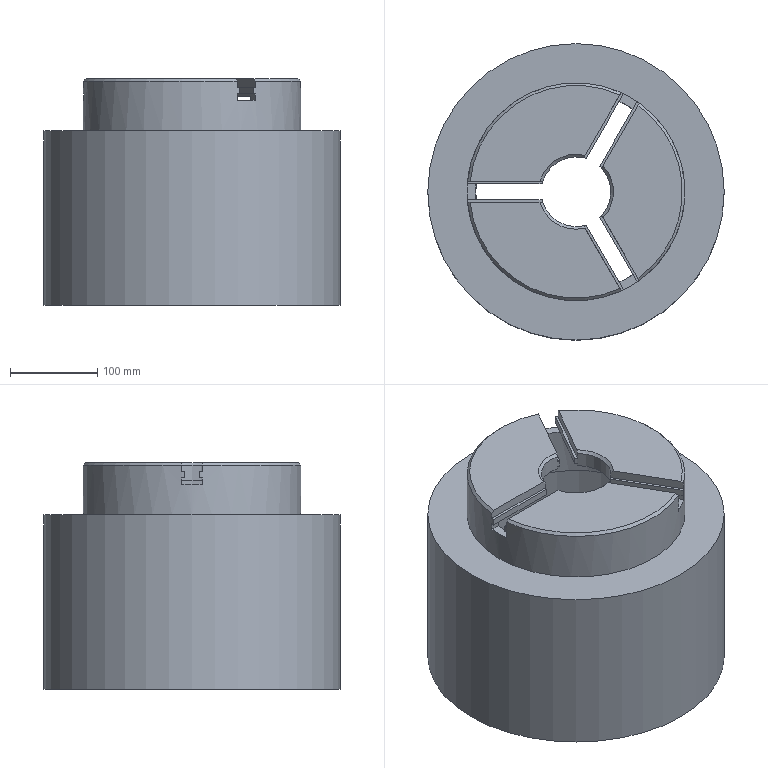Component | NX | CHUCK | 1 solid | 71 faces | volume 5662954 mm3 | plane 42 | cylinder 15 | cone 14 | commonest cylinder face diameters 6.8 x8 80 x3 340 x1 300 x1 230 x1 250 x1